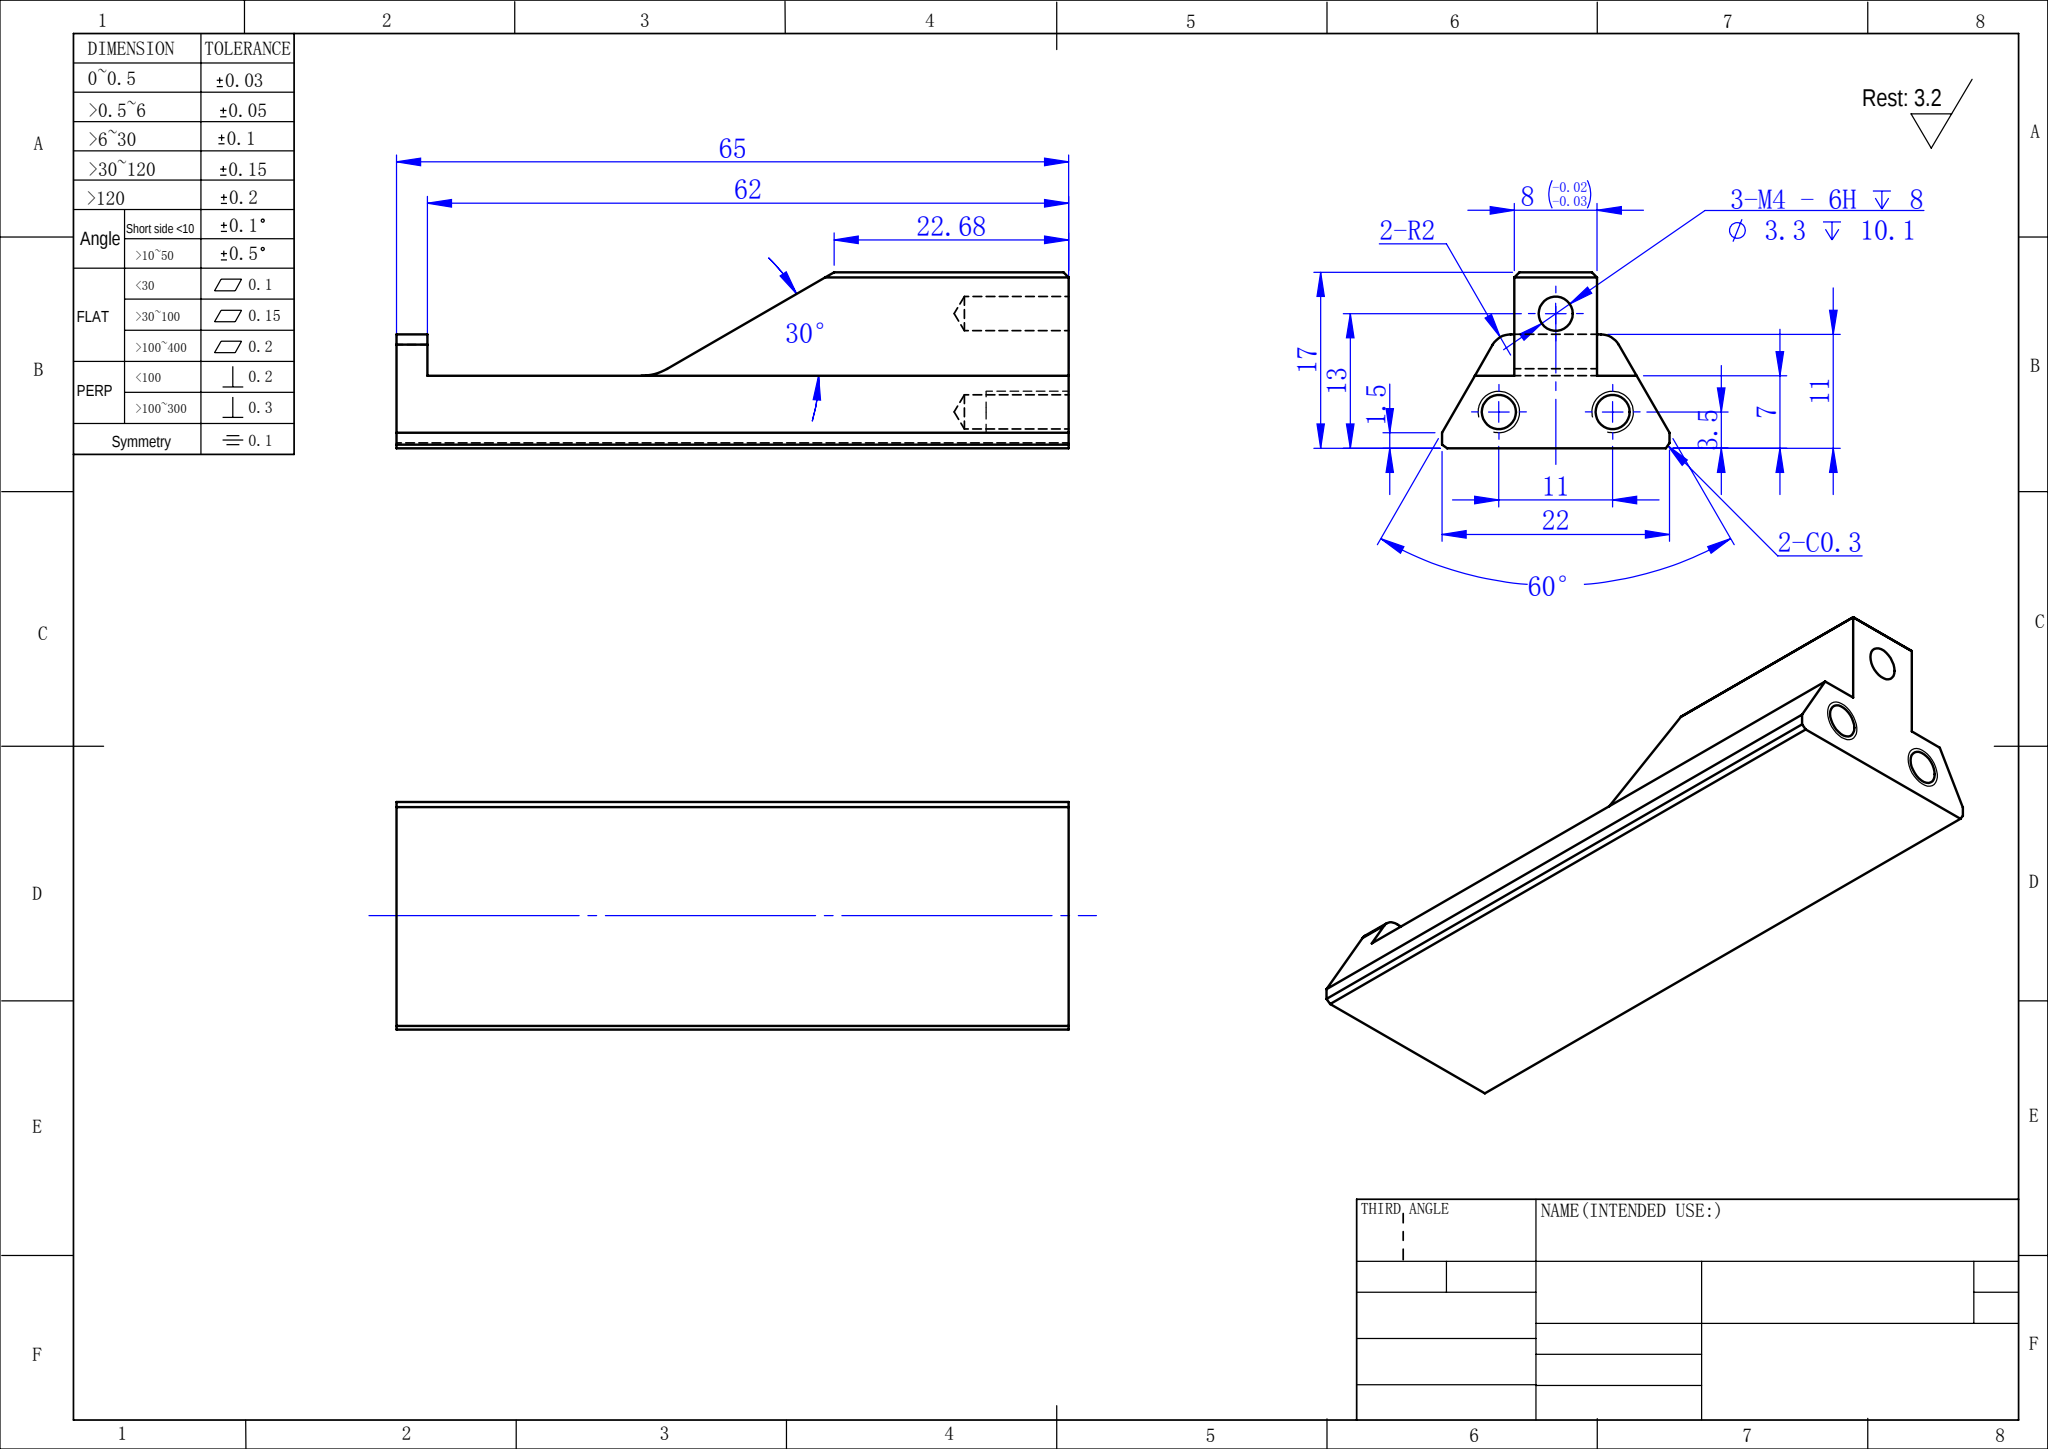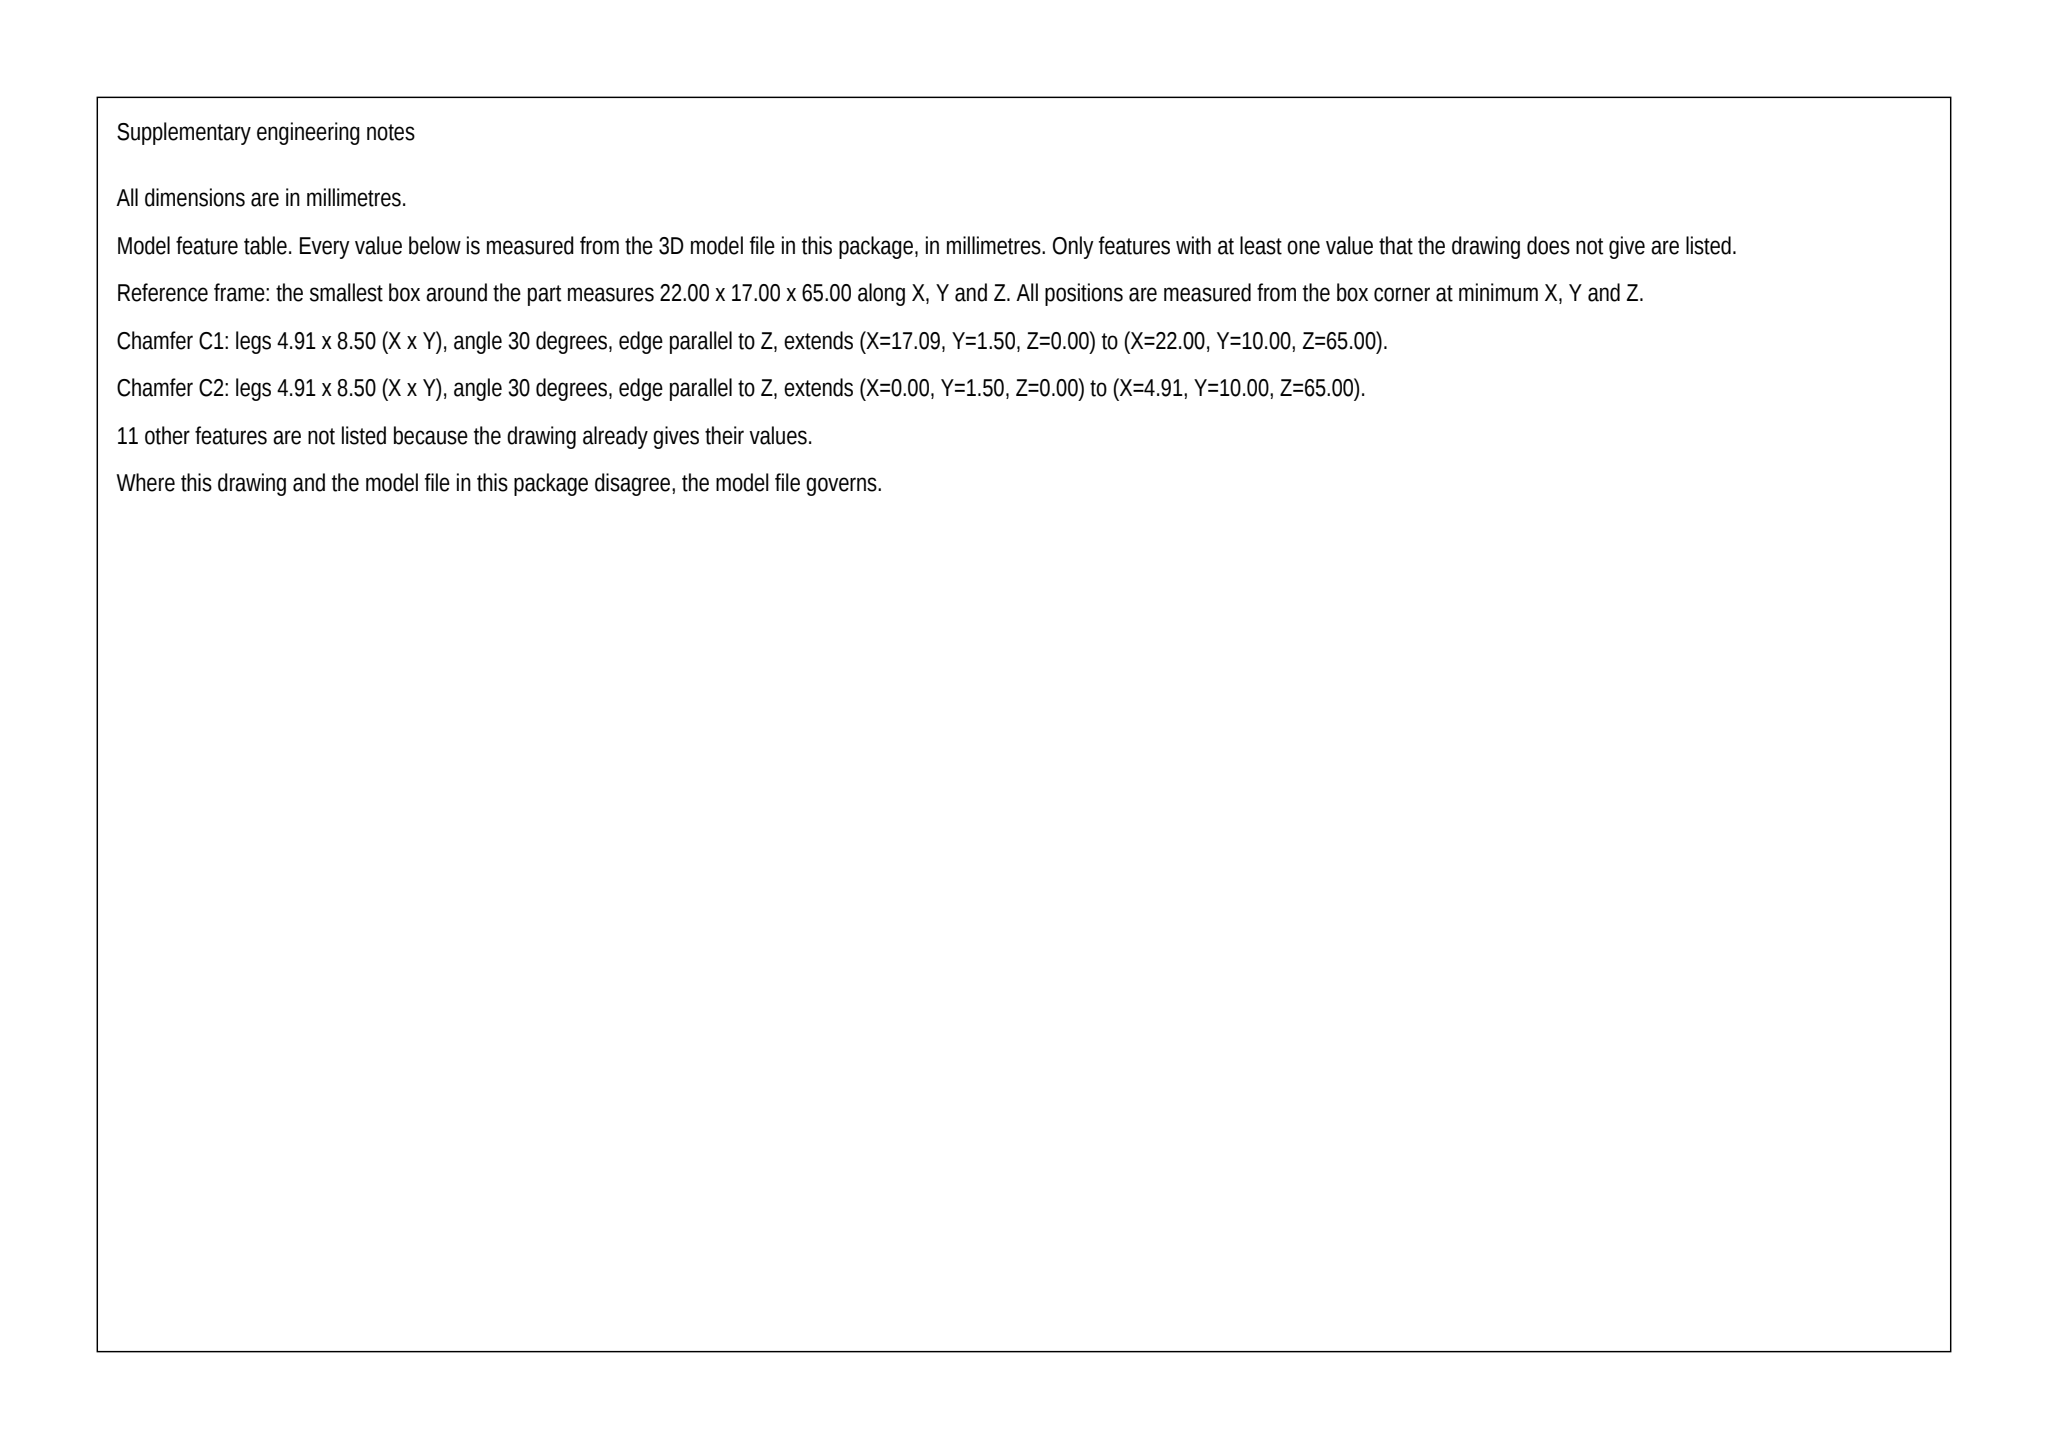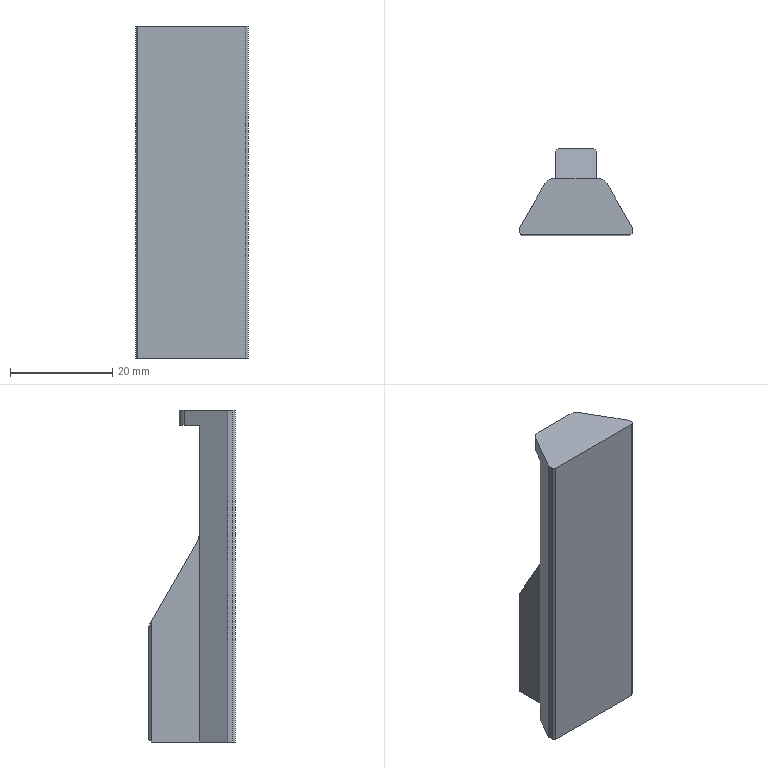Part | SolidWorks | mm | 1 solid | 34 faces | box 22 x 17 x 65 mm | volume 11256 mm3 | plane 19 | cylinder 9 | cone 6 | commonest cylinder face diameters 3.3 x6 4 x2 10 x1
build123d program:
from build123d import *
from OCP.BRepFilletAPI import BRepFilletAPI_MakeChamfer

# Parameters (mm, degrees)
BOSS_EXTRUDE1_DEPTH      = 65
SKETCH3_W                = 16
SKETCH3_H                = 3
BOSS_EXTRUDE2_DEPTH      = 4
M4_TAPPED_HOLE1_D        = 3.3
M4_TAPPED_HOLE1_DEPTH    = 10.1
M4_TAPPED_HOLE1_TIP      = 0.9914
CHAMFER2_SIZE            = 0.5
CHAMFER2_SIZE2           = 0.3501
CUT_EXTRUDE2_DEPTH       = 10
FILLET1_R                = 2
BOSS_EXTRUDE4_DEPTH      = 4
BOSS_EXTRUDE4_DEPTH_BACK = 4
M4_TAPPED_HOLE2_D        = 3.3
M4_TAPPED_HOLE2_DEPTH    = 10.1
M4_TAPPED_HOLE2_TIP      = 0.9914
FILLET2_R                = 5
CHAMFER3_SIZE            = 0.5


with BuildPart() as part:
    # Sketch1 → Boss-Extrude1 (new body)
    with BuildSketch(Plane.XY):
        Polygon((-11, 0), (-11, 1.5), (-7.825, 7), (7.825, 7), (11, 1.5), (11, 0), align=None)
    extrude(amount=BOSS_EXTRUDE1_DEPTH)

    # Sketch3 → Boss-Extrude2 (add)
    with BuildSketch(Plane(origin=(0, 7, 0), x_dir=(1, 0, 0), z_dir=(0, 1, 0))):
        with Locations((0, -63.5)):
            Rectangle(SKETCH3_W, SKETCH3_H)
    extrude(amount=BOSS_EXTRUDE2_DEPTH)

    # M4 Tapped Hole1
    with Locations(Plane(origin=(0, 0, 0), x_dir=(-1, 0, 0), z_dir=(0, 0, -1))):
        with Locations((5.5, 3.5), (-5.5, 3.5)):
            Hole(M4_TAPPED_HOLE1_D / 2, depth=M4_TAPPED_HOLE1_DEPTH)
            with Locations((0, 0, -(M4_TAPPED_HOLE1_DEPTH + M4_TAPPED_HOLE1_TIP / 2))):  # 118° drill point
                Cone(0, M4_TAPPED_HOLE1_D / 2, M4_TAPPED_HOLE1_TIP, mode=Mode.SUBTRACT)

    # Chamfer2: one chamfer whose edges measure the first distance from different faces: ONE call of the kernel's chamfer builder (chamfer() names one face for all edges)
    chamfer2_edges_1 = [part.edges().sort_by_distance(p)[0] for p in [
        (-11, 0, 32.5),
    ]]
    chamfer2_side_1 = [part.faces().sort_by_distance(p)[0] for p in [
        (-11, 0.75, 32.5),
    ]]
    chamfer2_edges_2 = [part.edges().sort_by_distance(p)[0] for p in [
        (11, 0, 32.5),
    ]]
    chamfer2_side_2 = [part.faces().sort_by_distance(p)[0] for p in [
        (0, 0, 32.5),
    ]]
    chamfer2 = BRepFilletAPI_MakeChamfer(part.part.solid().wrapped)
    for e in chamfer2_edges_1:
        chamfer2.Add(CHAMFER2_SIZE, CHAMFER2_SIZE2, e.wrapped, chamfer2_side_1[0].wrapped)  # the first distance lies on this face
    for e in chamfer2_edges_2:
        chamfer2.Add(CHAMFER2_SIZE, CHAMFER2_SIZE2, e.wrapped, chamfer2_side_2[0].wrapped)  # the first distance lies on this face
    add(Compound.cast(chamfer2.Shape()), mode=Mode.REPLACE)

    # Sketch11 → Cut-Extrude2 (cut)
    with BuildSketch(Plane.XY.offset(65)):
        Polygon((-8.553, 5.738), (-5.515, 11), (-8, 11), align=None)
        Polygon((8.459, 5.901), (5.515, 11), (8.936, 11), align=None)
    extrude(amount=-CUT_EXTRUDE2_DEPTH, mode=Mode.SUBTRACT)

    # Fillet1
    fillet1_edges = [part.edges().sort_by_distance(p)[0] for p in [
        (5.515, 11, 63.5),
        (-5.515, 11, 63.5),
    ]]
    fillet(fillet1_edges, radius=FILLET1_R)

    # Sketch13 → Boss-Extrude4 (add, two sides: drawn at the far end of the back side and taken through both)
    with BuildSketch(Plane(origin=(0, 0, 0), x_dir=(0, 0, -1), z_dir=(1, 0, 0)).offset(-BOSS_EXTRUDE4_DEPTH_BACK)):
        Polygon((0, 7), (0, 17), (-22.679, 17), (-40, 7), align=None)
    extrude(amount=BOSS_EXTRUDE4_DEPTH + BOSS_EXTRUDE4_DEPTH_BACK)

    # M4 Tapped Hole2
    with Locations(Plane(origin=(0, 0, 0), x_dir=(-1, 0, 0), z_dir=(0, 0, -1))):
        with Locations((0, 13)):
            Hole(M4_TAPPED_HOLE2_D / 2, depth=M4_TAPPED_HOLE2_DEPTH)
            with Locations((0, 0, -(M4_TAPPED_HOLE2_DEPTH + M4_TAPPED_HOLE2_TIP / 2))):  # 118° drill point
                Cone(0, M4_TAPPED_HOLE2_D / 2, M4_TAPPED_HOLE2_TIP, mode=Mode.SUBTRACT)

    # Fillet2
    fillet2_edges = [part.edges().sort_by_distance(p)[0] for p in [
        (0, 7, 40),
    ]]
    fillet(fillet2_edges, radius=FILLET2_R)

    # Chamfer3
    chamfer3_edges = [part.edges().sort_by_distance(p)[0] for p in [
        (-4, 17, 11.34),
        (0, 17, 0),
        (4, 17, 11.34),
    ]]
    chamfer(chamfer3_edges, length=CHAMFER3_SIZE)


solid = part.part